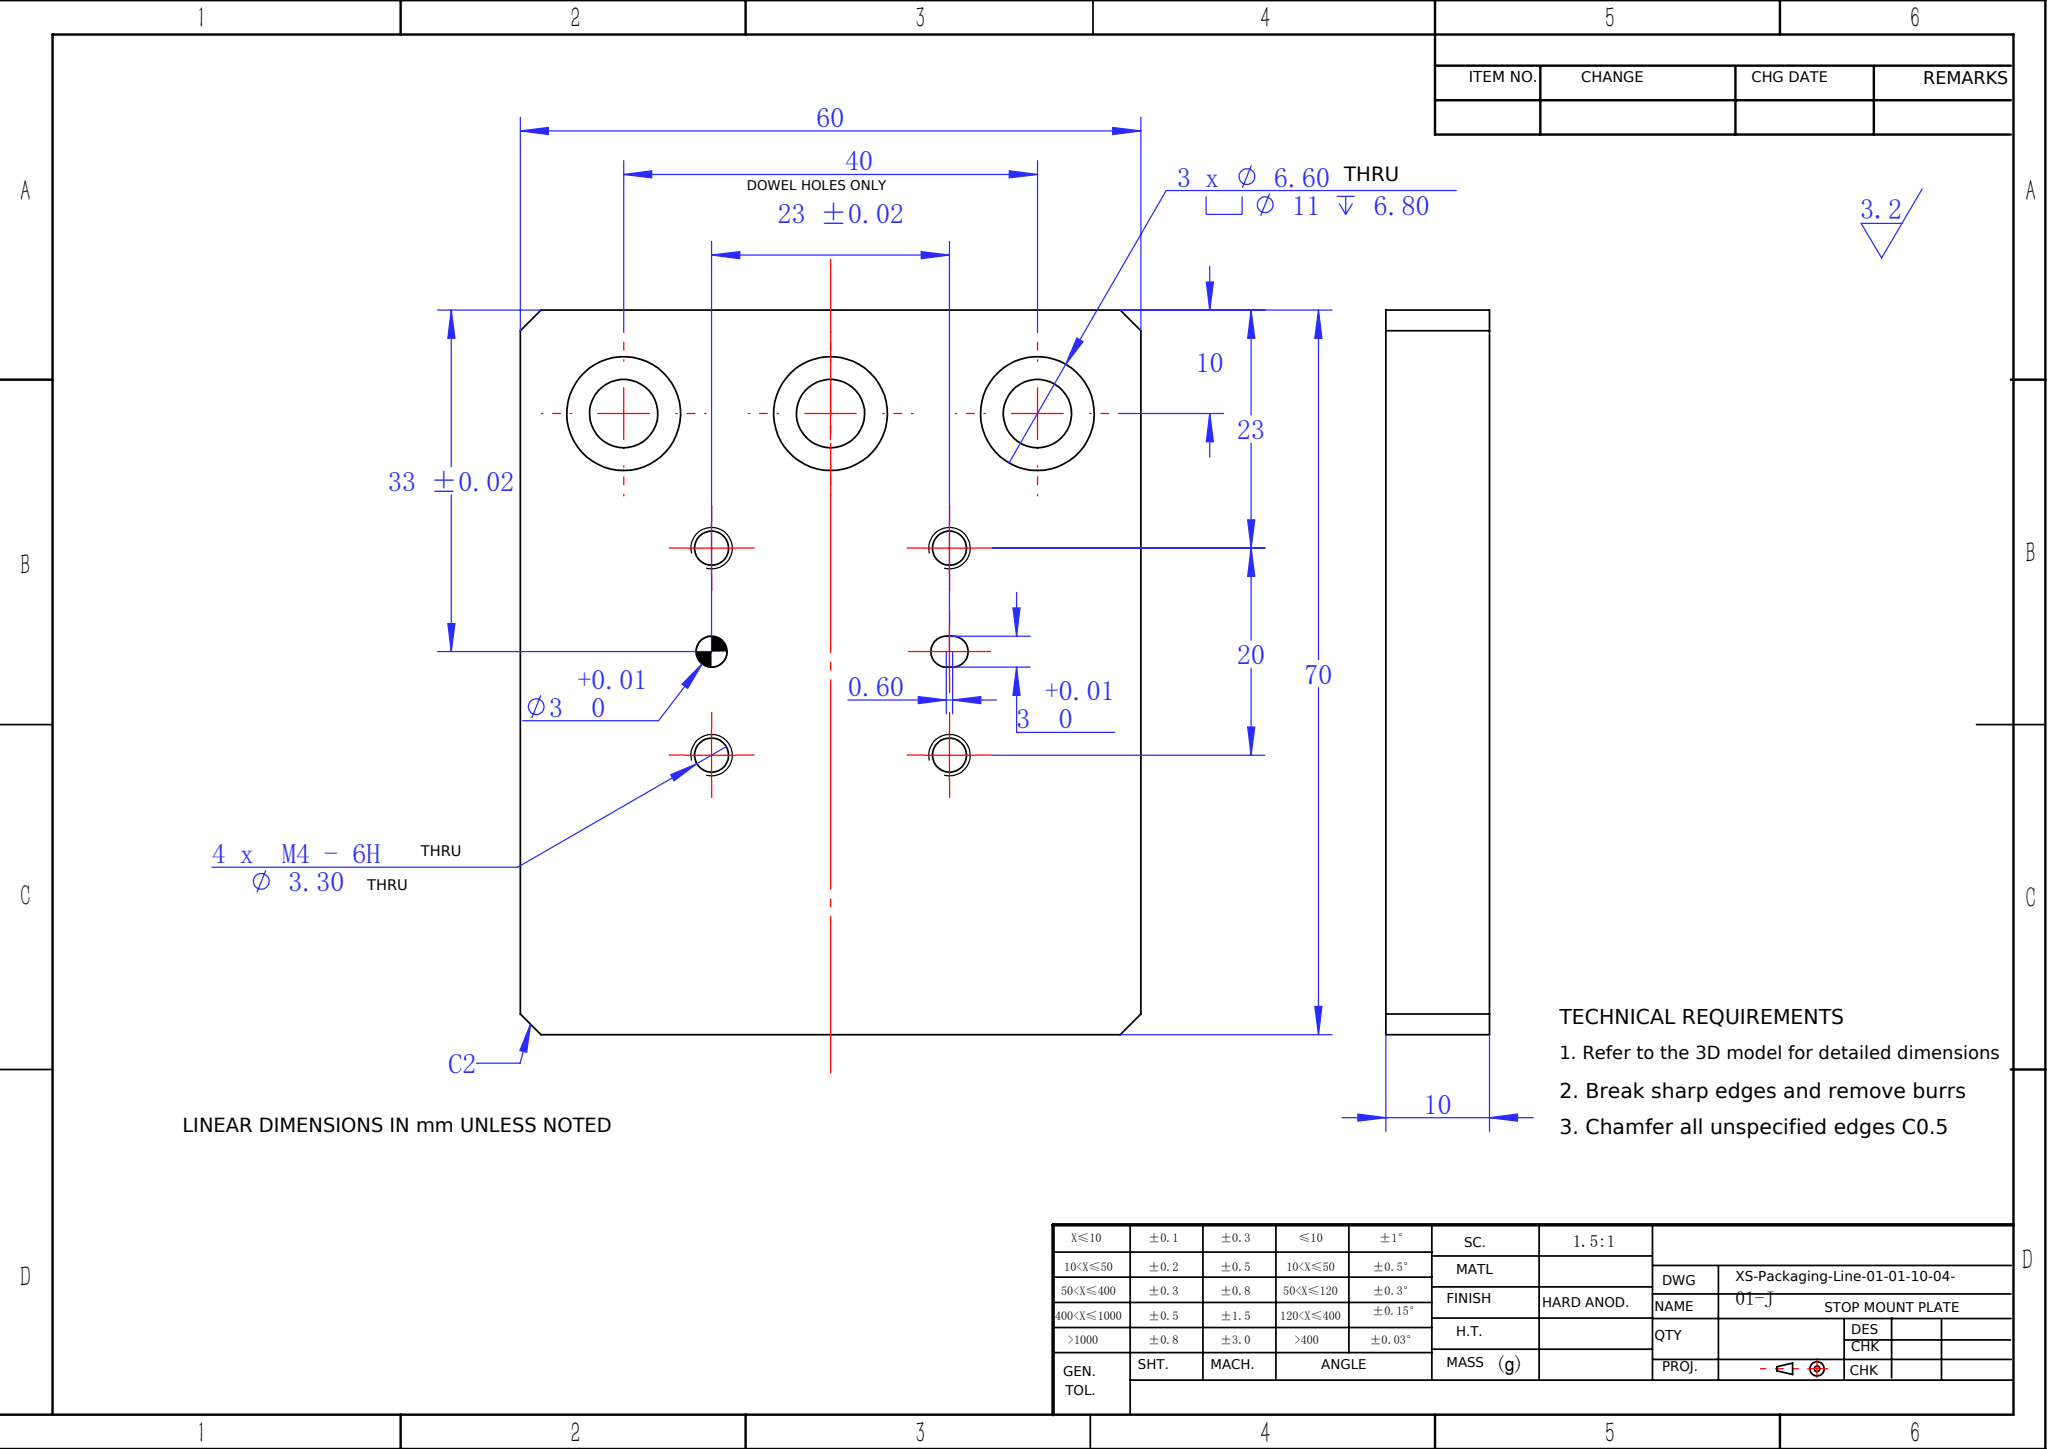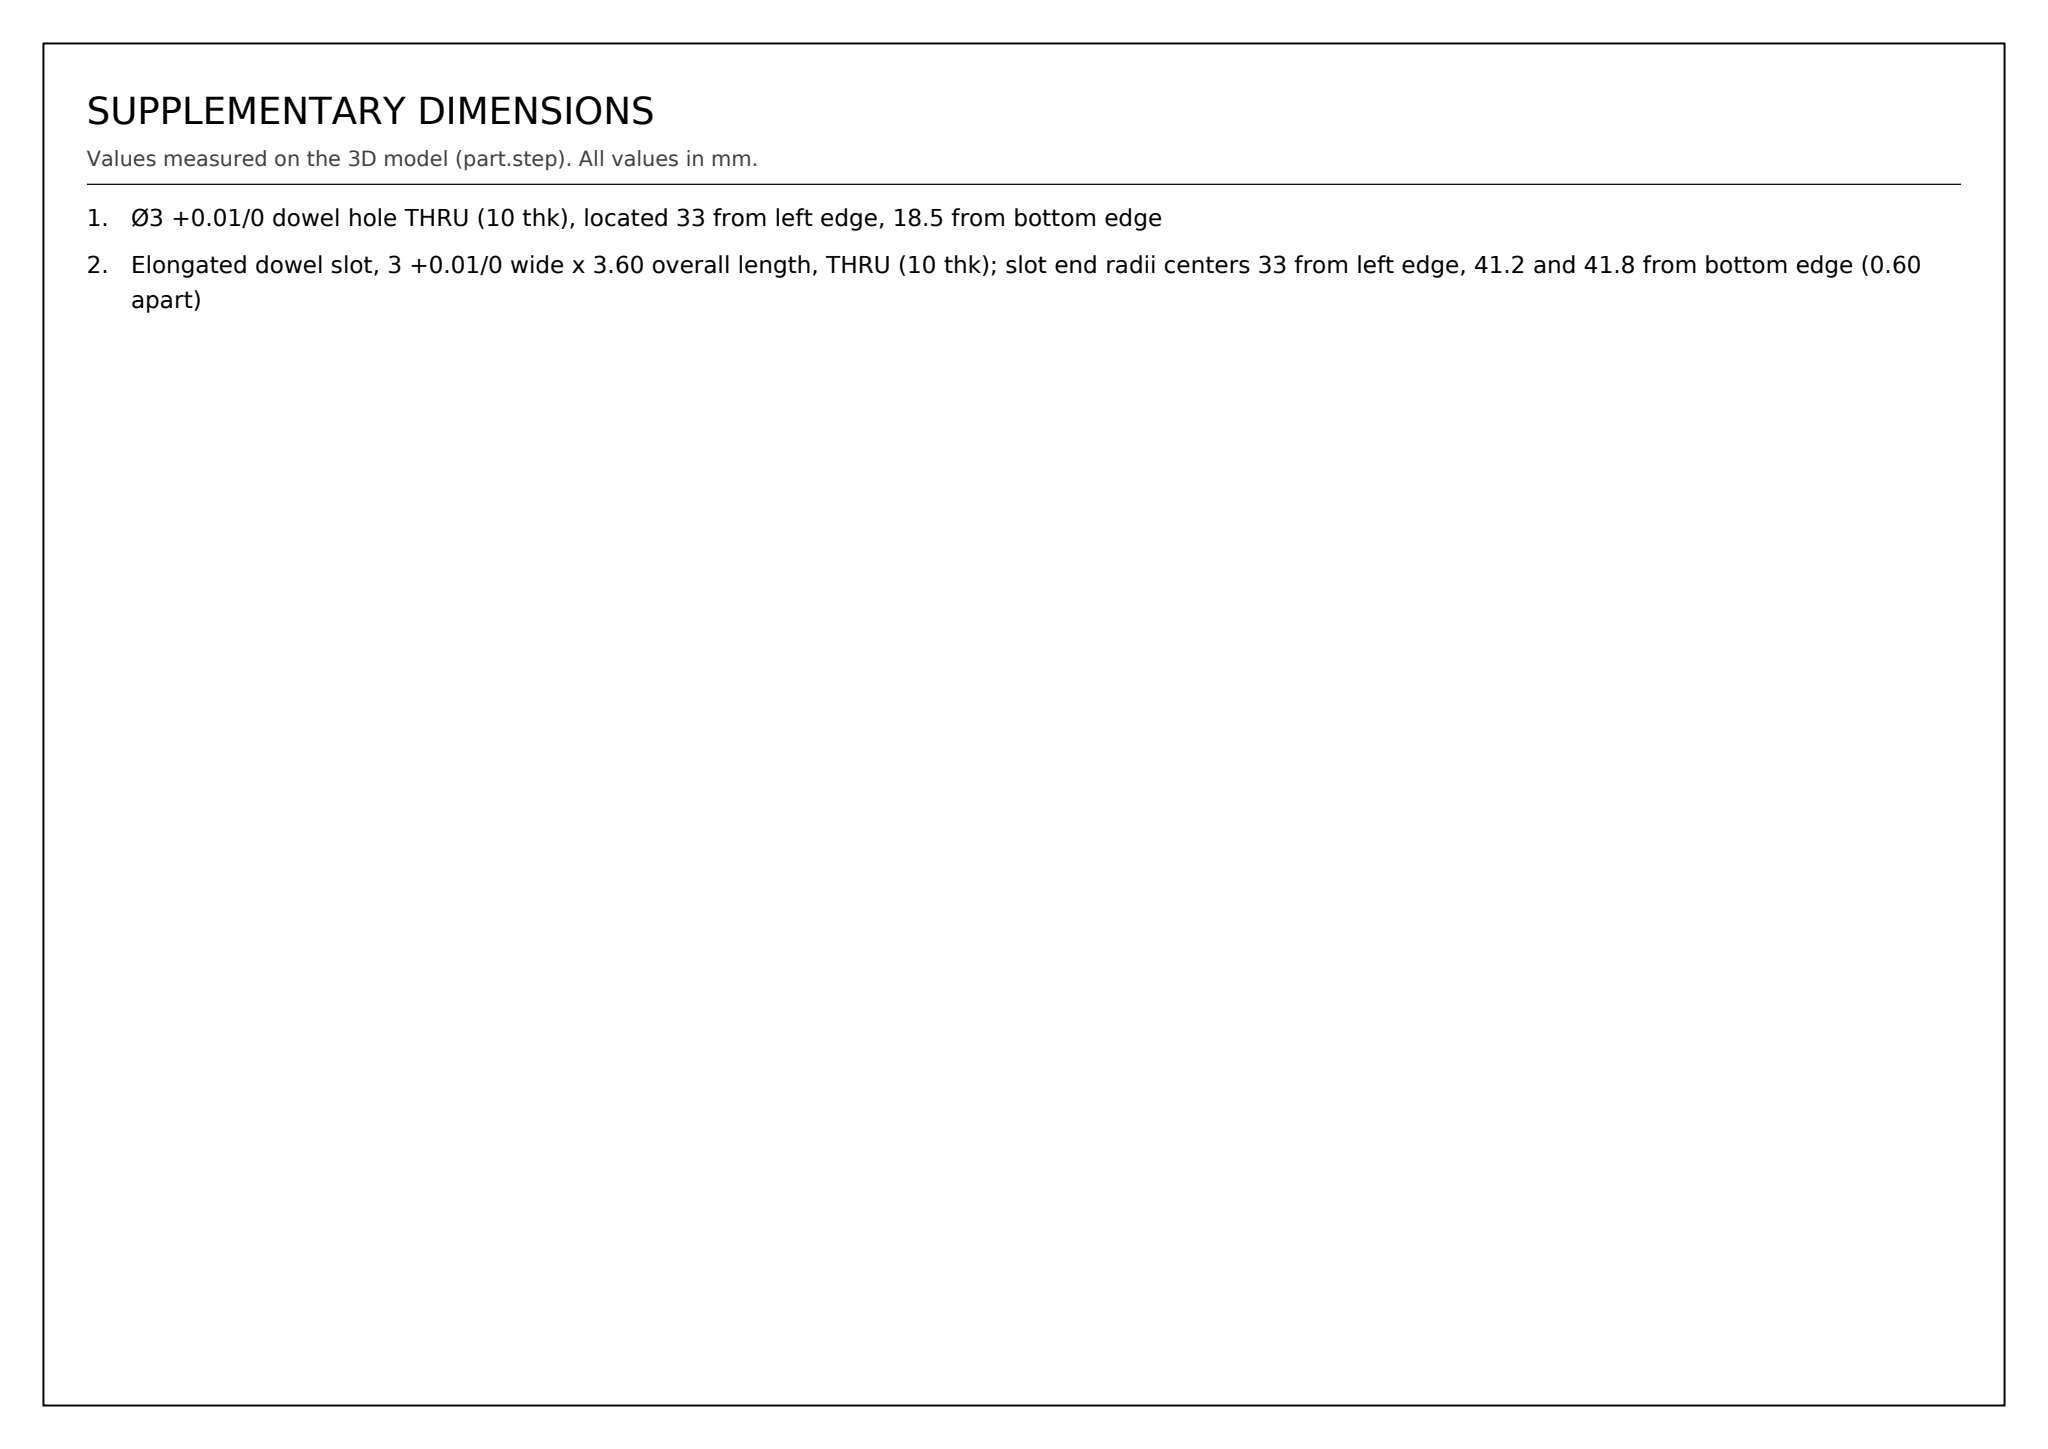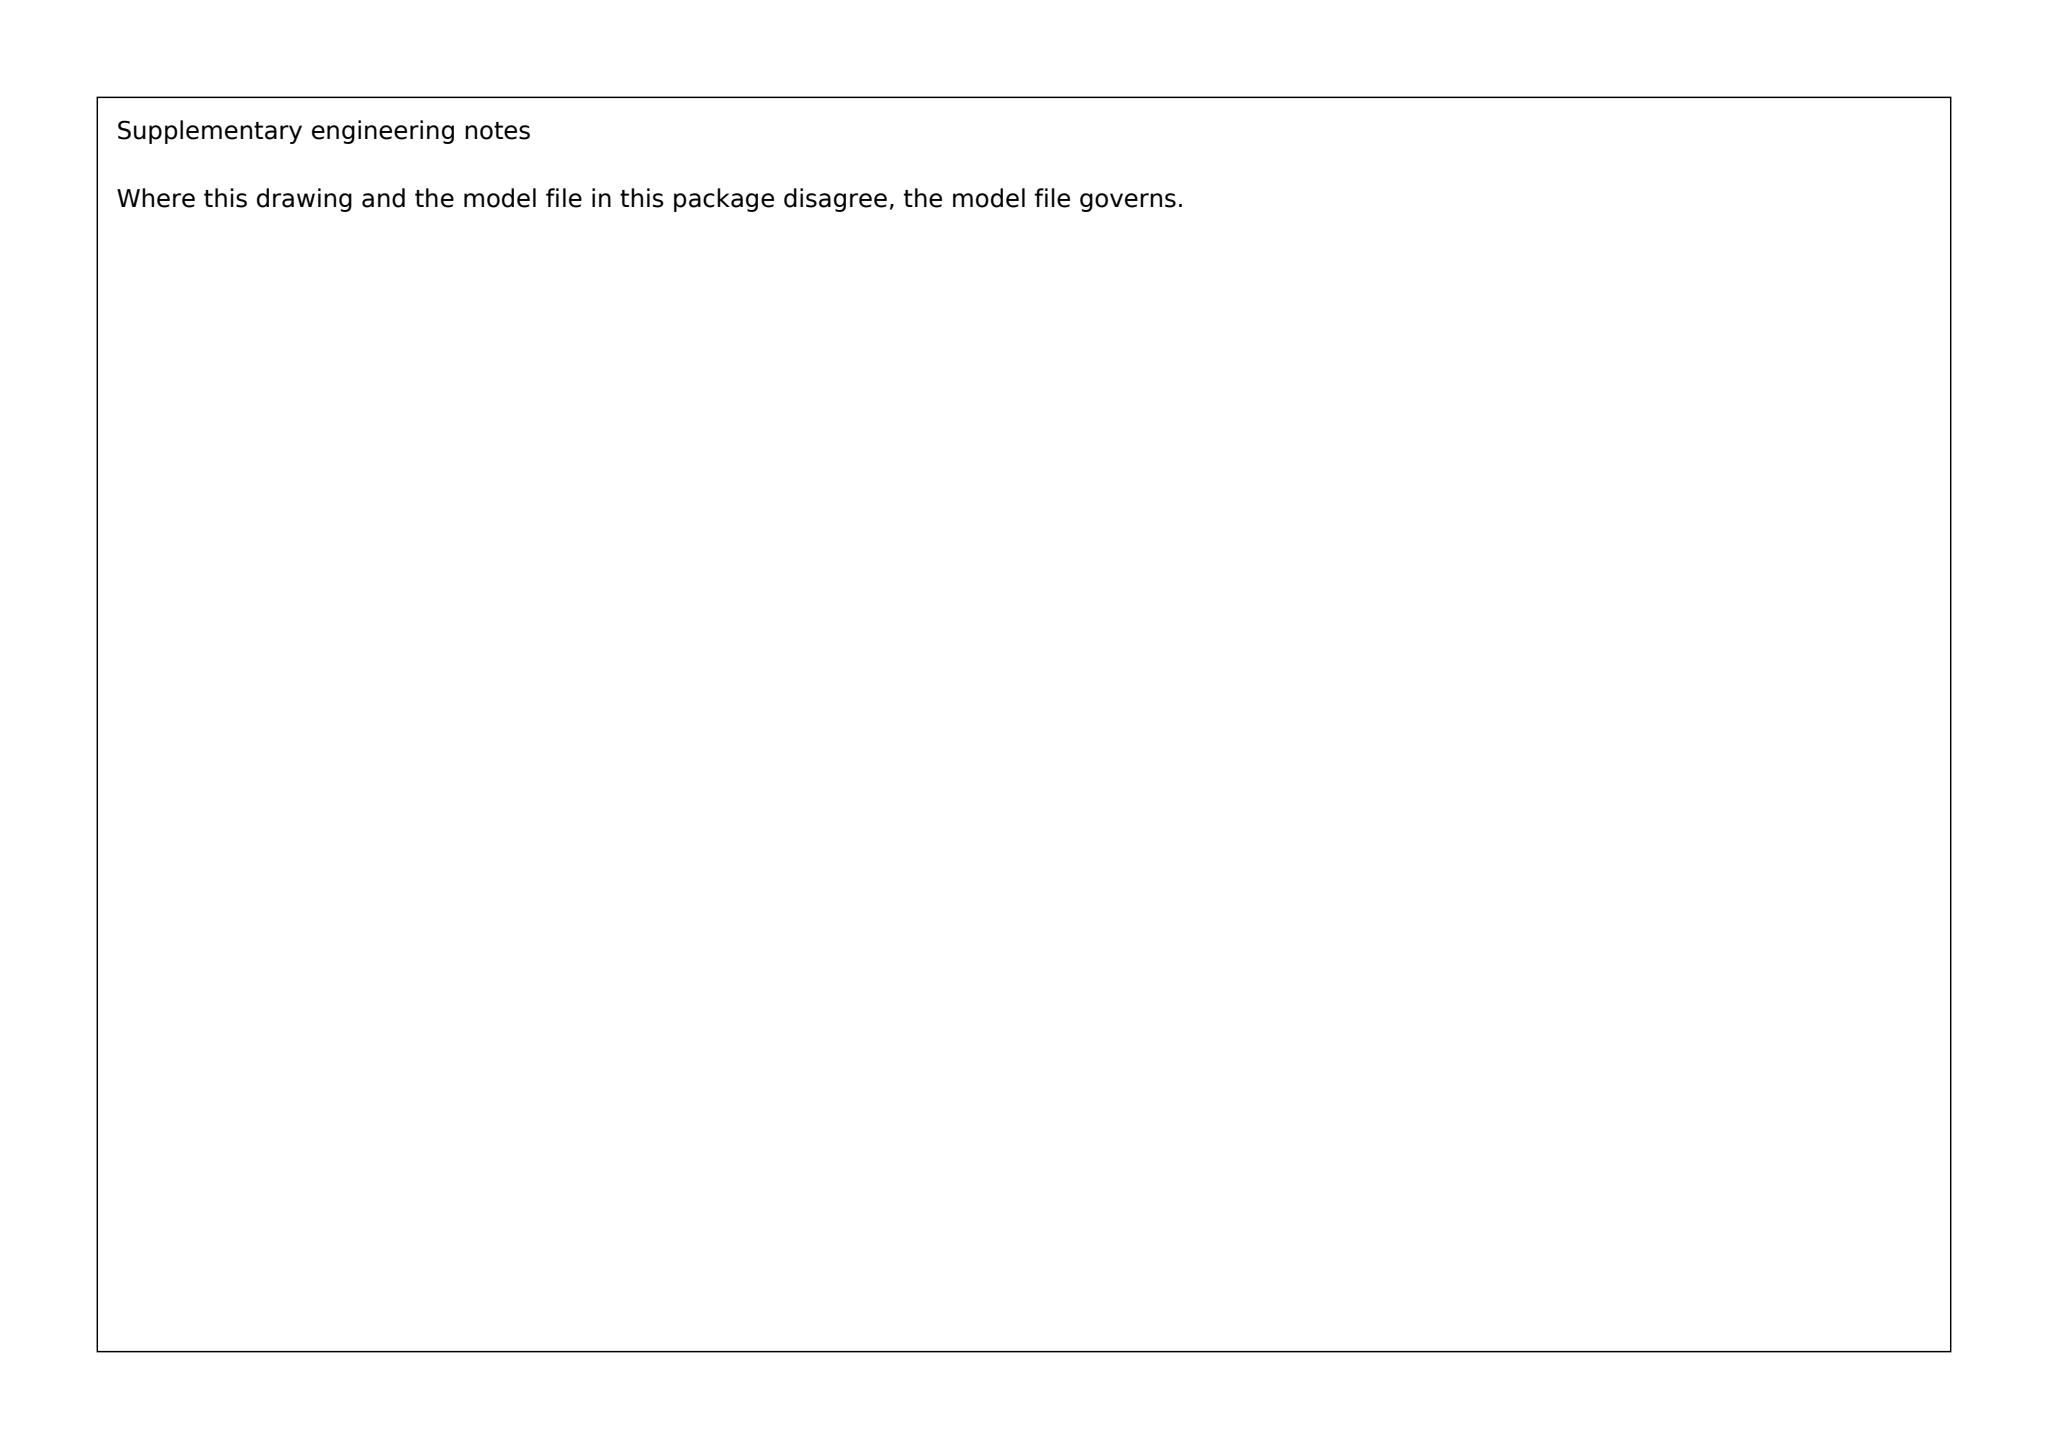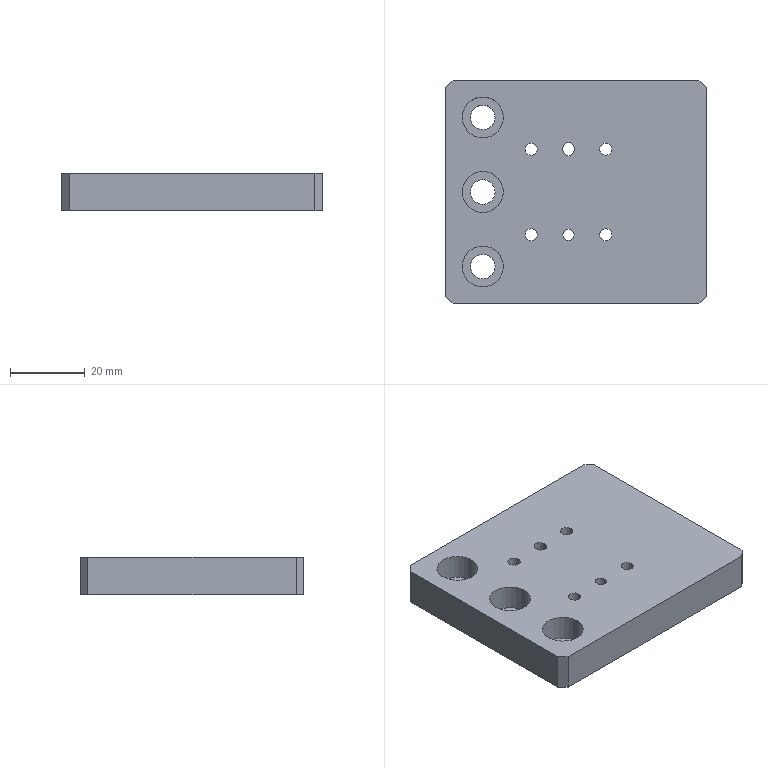Part | SolidWorks | mm | 1 solid | 44 faces | box 70 x 60 x 10 mm | volume 39151 mm3 | cylinder 31 | plane 13 | commonest cylinder face diameters 3 x11 3.3 x8 11 x6 6.6 x6
Drawing notes:
Ø3 +0.01/0 dowel hole THRU (10 thk), located 33 from left edge, 18.5 from bottom edge | from the solid: cylinders: hole/bore dia 3.0, axis z at [33.0, 18.5], from 0.0 to 10.0, 360 deg; bbox_xyz Z=10
Elongated dowel slot, 3 +0.01/0 wide x 3.60 overall length, THRU (10 thk); slot end radii centers 33 from left edge, 41.2 and 41.8 from bottom edge (0.60 apart) | from the solid: cylinders: concave arcs dia 3.0, axis z at [33.0, 41.2] and [33.0, 41.8], each from 0.0 to 10.0, 191 deg; bbox_xyz Z=10
build123d program:
from build123d import *

# Parameters (mm, degrees)
SKETCH1_W                                       = 70
SKETCH1_H                                       = 60
BOSS_EXTRUDE1_DEPTH                             = 10
M4_TAPPED_HOLE1_D                               = 3.3
F_3_0MM_DOWEL_PIN_HOLE_1_D                      = 3
M6_HEX_SOCKET_HEAD_CAP_SCREW_CBORE1_D           = 6.6
M6_HEX_SOCKET_HEAD_CAP_SCREW_CBORE1_CBORE_D     = 11
M6_HEX_SOCKET_HEAD_CAP_SCREW_CBORE1_CBORE_DEPTH = 6.8
CHAMFER1_SIZE                                   = 2


with BuildPart() as part:
    # Sketch1 → Boss-Extrude1 (new body)
    with BuildSketch(Plane.XY):
        Rectangle(SKETCH1_W, SKETCH1_H)
    extrude(amount=BOSS_EXTRUDE1_DEPTH)

    # M4 Tapped Hole1 (through all)
    with Locations(Plane.XY.offset(10)):
        with Locations((-12, -11.5), (8, -11.5), (8, 11.5), (-12, 11.5)):
            Hole(M4_TAPPED_HOLE1_D / 2)

    # 3.0mm Dowel Pin Hole 1 (through all)
    with Locations(Plane(origin=(0, 0, 0), x_dir=(-1, 0, 0), z_dir=(0, 0, -1))):
        with Locations((2, 11.5), (2, -11.5), (2, 11.2), (2, 11.8)):
            Hole(F_3_0MM_DOWEL_PIN_HOLE_1_D / 2)

    # M6 Hex Socket Head Cap Screw CBORE1 (through all)
    with Locations(Plane.XY.offset(10)):
        with Locations((-25, -20), (-25, 0), (-25, 20)):
            CounterBoreHole(M6_HEX_SOCKET_HEAD_CAP_SCREW_CBORE1_D / 2, M6_HEX_SOCKET_HEAD_CAP_SCREW_CBORE1_CBORE_D / 2, M6_HEX_SOCKET_HEAD_CAP_SCREW_CBORE1_CBORE_DEPTH)

    # Chamfer1
    chamfer1_edges = [part.edges().sort_by_distance(p)[0] for p in [
        (35, -30, 5),
        (-35, -30, 5),
        (-35, 30, 5),
        (35, 30, 5),
    ]]
    chamfer(chamfer1_edges, length=CHAMFER1_SIZE)


solid = part.part